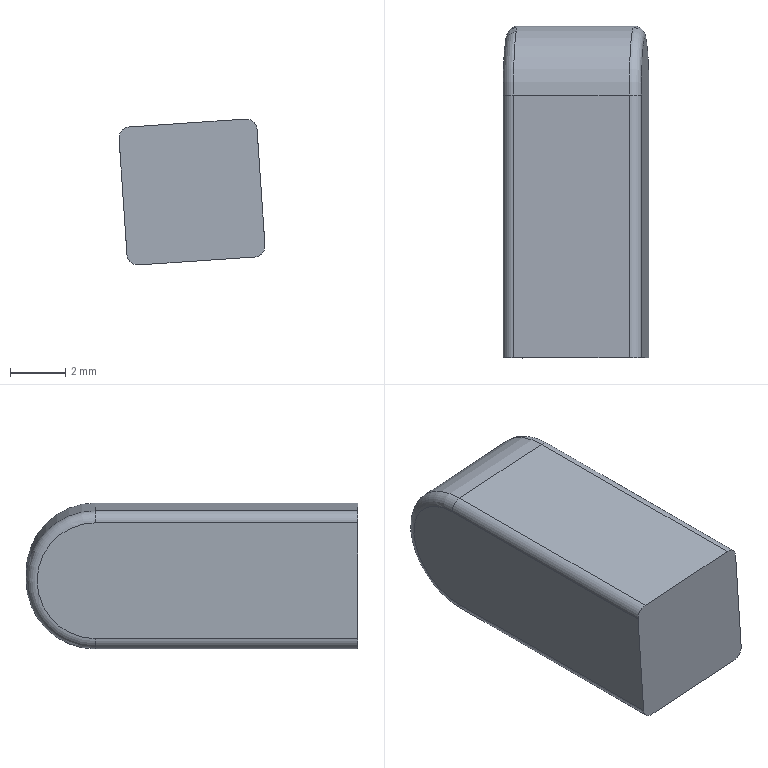Component | SolidWorks | GB_T1096-1979PlainParallelKeyC-type5_12-2 | 1 solid | 13 faces | box 5.28 x 12 x 5.28 mm | volume 285 mm3 | cylinder 6 | plane 5 | torus 2 | commonest cylinder face diameters 0.8 x4 5 x2
build123d program:
from build123d import *

# Parameters (mm, degrees)
BASE_EXTRUDE_DEPTH = 5
FILLET1_R          = 0.4


with BuildPart() as part:
    # Sketch1 → Base-Extrude (new body)
    with BuildSketch(Plane.XY):
        with BuildLine():
            Line((-9, 2.5), (0.5, 2.5))
            Line((0.5, 2.5), (0.5, -2.5))
            Line((0.5, -2.5), (-9, -2.5))
            ThreePointArc((-9, -2.5), (-11.5, 0), (-9, 2.5))
        make_face()
    extrude(amount=BASE_EXTRUDE_DEPTH)

    # Fillet1
    fillet1_edges = [part.edges().sort_by_distance(p)[0] for p in [
        (-11.5, 0, 5),
        (-4.25, -2.5, 5),
        (-4.25, -2.5, 0),
        (-11.5, 0, 0),
        (-4.25, 2.5, 0),
        (-4.25, 2.5, 5),
    ]]
    fillet(fillet1_edges, radius=FILLET1_R)


solid = part.part

# Placed as in the assembly
solid = solid.moved(Location((-17.866, 61.766, -165.86), (180, -86.093, 90)))
STEP:
#1=COLOUR_RGB('',0.7922,0.8196,0.9333);
#2=FILL_AREA_STYLE_COLOUR('',#1);
#3=FILL_AREA_STYLE('',(#2));
#4=SURFACE_STYLE_FILL_AREA(#3);
#5=SURFACE_SIDE_STYLE('',(#4));
#6=SURFACE_STYLE_USAGE(.BOTH.,#5);
#7=PRESENTATION_STYLE_ASSIGNMENT((#6));
#8=CARTESIAN_POINT('',(-0.8774,2.786,-6.64));
#9=VERTEX_POINT('',#8);
#10=CARTESIAN_POINT('',(-0.8841,2.884,-6.542));
#11=VERTEX_POINT('',#10);
#12=CARTESIAN_POINT('',(-0.8841,2.786,-6.542));
#13=DIRECTION('',(0.9977,0.,0.06814));
#14=DIRECTION('',(0.,-1.,0.));
#15=AXIS2_PLACEMENT_3D('',#12,#13,#14);
#16=CIRCLE('',#15,0.09843);
#17=EDGE_CURVE('',#9,#11,#16,.T.);
#18=ORIENTED_EDGE('',*,*,#17,.T.);
#19=CARTESIAN_POINT('',(-0.7191,2.884,-6.531));
#20=VERTEX_POINT('',#19);
#21=CARTESIAN_POINT('',(-0.8998,2.884,-6.543));
#22=DIRECTION('',(0.9977,0.,0.06814));
#23=VECTOR('',#22,39.37);
#24=LINE('',#21,#23);
#25=EDGE_CURVE('',#11,#20,#24,.T.);
#26=ORIENTED_EDGE('',*,*,#25,.T.);
#27=CARTESIAN_POINT('',(-0.7124,2.786,-6.629));
#28=VERTEX_POINT('',#27);
#29=CARTESIAN_POINT('',(-0.7191,2.786,-6.531));
#30=DIRECTION('',(-0.9977,-0.,-0.06814));
#31=DIRECTION('',(0.,-1.,0.));
#32=AXIS2_PLACEMENT_3D('',#29,#30,#31);
#33=CIRCLE('',#32,0.09843);
#34=EDGE_CURVE('',#20,#28,#33,.T.);
#35=ORIENTED_EDGE('',*,*,#34,.T.);
#36=CARTESIAN_POINT('',(-0.8931,2.786,-6.642));
#37=DIRECTION('',(0.9977,0.,0.06814));
#38=VECTOR('',#37,39.37);
#39=LINE('',#36,#38);
#40=EDGE_CURVE('',#9,#28,#39,.T.);
#41=ORIENTED_EDGE('',*,*,#40,.F.);
#42=EDGE_LOOP('',(#18,#26,#35,#41));
#43=FACE_OUTER_BOUND('',#42,.T.);
#44=CARTESIAN_POINT('',(-0.8998,2.786,-6.543));
#45=DIRECTION('',(0.9977,0.,0.06814));
#46=DIRECTION('',(0.,1.,0.));
#47=AXIS2_PLACEMENT_3D('',#44,#45,#46);
#48=CYLINDRICAL_SURFACE('',#47,0.09843);
#49=ADVANCED_FACE('',(#43),#48,.T.);
#50=CARTESIAN_POINT('',(-0.8942,2.412,-6.626));
#51=VERTEX_POINT('',#50);
#52=CARTESIAN_POINT('',(-0.9054,2.412,-6.461));
#53=VERTEX_POINT('',#52);
#54=CARTESIAN_POINT('',(-0.9065,2.412,-6.445));
#55=DIRECTION('',(-0.06814,0.,0.9977));
#56=VECTOR('',#55,39.37);
#57=LINE('',#54,#56);
#58=EDGE_CURVE('',#51,#53,#57,.T.);
#59=ORIENTED_EDGE('',*,*,#58,.F.);
#60=CARTESIAN_POINT('',(-0.8774,2.412,-6.64));
#61=VERTEX_POINT('',#60);
#62=CARTESIAN_POINT('',(-0.8785,2.412,-6.625));
#63=DIRECTION('',(0.,-1.,0.));
#64=DIRECTION('',(-0.9977,0.,-0.06814));
#65=AXIS2_PLACEMENT_3D('',#62,#63,#64);
#66=CIRCLE('',#65,0.01575);
#67=EDGE_CURVE('',#51,#61,#66,.T.);
#68=ORIENTED_EDGE('',*,*,#67,.T.);
#69=CARTESIAN_POINT('',(-0.7124,2.412,-6.629));
#70=VERTEX_POINT('',#69);
#71=CARTESIAN_POINT('',(-0.8931,2.412,-6.642));
#72=DIRECTION('',(0.9977,0.,0.06814));
#73=VECTOR('',#72,39.37);
#74=LINE('',#71,#73);
#75=EDGE_CURVE('',#61,#70,#74,.T.);
#76=ORIENTED_EDGE('',*,*,#75,.T.);
#77=CARTESIAN_POINT('',(-0.6978,2.412,-6.612));
#78=VERTEX_POINT('',#77);
#79=CARTESIAN_POINT('',(-0.7135,2.412,-6.613));
#80=DIRECTION('',(0.,-1.,0.));
#81=DIRECTION('',(-0.9977,0.,-0.06814));
#82=AXIS2_PLACEMENT_3D('',#79,#80,#81);
#83=CIRCLE('',#82,0.01575);
#84=EDGE_CURVE('',#70,#78,#83,.T.);
#85=ORIENTED_EDGE('',*,*,#84,.T.);
#86=CARTESIAN_POINT('',(-0.709,2.412,-6.447));
#87=VERTEX_POINT('',#86);
#88=CARTESIAN_POINT('',(-0.7101,2.412,-6.432));
#89=DIRECTION('',(-0.06814,0.,0.9977));
#90=VECTOR('',#89,39.37);
#91=LINE('',#88,#90);
#92=EDGE_CURVE('',#78,#87,#91,.T.);
#93=ORIENTED_EDGE('',*,*,#92,.T.);
#94=CARTESIAN_POINT('',(-0.7258,2.412,-6.433));
#95=VERTEX_POINT('',#94);
#96=CARTESIAN_POINT('',(-0.7247,2.412,-6.449));
#97=DIRECTION('',(0.,-1.,0.));
#98=DIRECTION('',(-0.9977,0.,-0.06814));
#99=AXIS2_PLACEMENT_3D('',#96,#97,#98);
#100=CIRCLE('',#99,0.01575);
#101=EDGE_CURVE('',#87,#95,#100,.T.);
#102=ORIENTED_EDGE('',*,*,#101,.T.);
#103=CARTESIAN_POINT('',(-0.8908,2.412,-6.444));
#104=VERTEX_POINT('',#103);
#105=CARTESIAN_POINT('',(-0.9065,2.412,-6.445));
#106=DIRECTION('',(0.9977,0.,0.06814));
#107=VECTOR('',#106,39.37);
#108=LINE('',#105,#107);
#109=EDGE_CURVE('',#104,#95,#108,.T.);
#110=ORIENTED_EDGE('',*,*,#109,.F.);
#111=CARTESIAN_POINT('',(-0.8897,2.412,-6.46));
#112=DIRECTION('',(0.,-1.,0.));
#113=DIRECTION('',(-0.9977,0.,-0.06814));
#114=AXIS2_PLACEMENT_3D('',#111,#112,#113);
#115=CIRCLE('',#114,0.01575);
#116=EDGE_CURVE('',#104,#53,#115,.T.);
#117=ORIENTED_EDGE('',*,*,#116,.T.);
#118=EDGE_LOOP('',(#59,#68,#76,#85,#93,#102,#110,#117));
#119=FACE_OUTER_BOUND('',#118,.T.);
#120=CARTESIAN_POINT('',(-0.9065,2.412,-6.445));
#121=DIRECTION('',(-0.,1.,-0.));
#122=DIRECTION('',(-0.9977,-0.,-0.06814));
#123=AXIS2_PLACEMENT_3D('',#120,#121,#122);
#124=PLANE('',#123);
#125=ADVANCED_FACE('',(#119),#124,.F.);
#126=CARTESIAN_POINT('',(-0.8908,2.786,-6.444));
#127=VERTEX_POINT('',#126);
#128=CARTESIAN_POINT('',(-0.7258,2.786,-6.433));
#129=VERTEX_POINT('',#128);
#130=CARTESIAN_POINT('',(-0.9065,2.786,-6.445));
#131=DIRECTION('',(0.9977,0.,0.06814));
#132=VECTOR('',#131,39.37);
#133=LINE('',#130,#132);
#134=EDGE_CURVE('',#127,#129,#133,.T.);
#135=ORIENTED_EDGE('',*,*,#134,.F.);
#136=CARTESIAN_POINT('',(-0.8908,2.412,-6.444));
#137=DIRECTION('',(0.,-1.,0.));
#138=VECTOR('',#137,39.37);
#139=LINE('',#136,#138);
#140=EDGE_CURVE('',#127,#104,#139,.T.);
#141=ORIENTED_EDGE('',*,*,#140,.T.);
#142=ORIENTED_EDGE('',*,*,#109,.T.);
#143=CARTESIAN_POINT('',(-0.7258,2.786,-6.433));
#144=DIRECTION('',(-0.,1.,-0.));
#145=VECTOR('',#144,39.37);
#146=LINE('',#143,#145);
#147=EDGE_CURVE('',#95,#129,#146,.T.);
#148=ORIENTED_EDGE('',*,*,#147,.T.);
#149=EDGE_LOOP('',(#135,#141,#142,#148));
#150=FACE_OUTER_BOUND('',#149,.T.);
#151=CARTESIAN_POINT('',(-0.9065,2.786,-6.445));
#152=DIRECTION('',(0.06814,-0.,-0.9977));
#153=DIRECTION('',(0.9977,0.,0.06814));
#154=AXIS2_PLACEMENT_3D('',#151,#152,#153);
#155=PLANE('',#154);
#156=ADVANCED_FACE('',(#150),#155,.F.);
#157=ORIENTED_EDGE('',*,*,#25,.F.);
#158=CARTESIAN_POINT('',(-0.8841,2.786,-6.542));
#159=DIRECTION('',(0.9977,0.,0.06814));
#160=DIRECTION('',(0.,-1.,0.));
#161=AXIS2_PLACEMENT_3D('',#158,#159,#160);
#162=CIRCLE('',#161,0.09843);
#163=EDGE_CURVE('',#11,#127,#162,.T.);
#164=ORIENTED_EDGE('',*,*,#163,.T.);
#165=ORIENTED_EDGE('',*,*,#134,.T.);
#166=CARTESIAN_POINT('',(-0.7191,2.786,-6.531));
#167=DIRECTION('',(-0.9977,-0.,-0.06814));
#168=DIRECTION('',(0.,-1.,0.));
#169=AXIS2_PLACEMENT_3D('',#166,#167,#168);
#170=CIRCLE('',#169,0.09843);
#171=EDGE_CURVE('',#129,#20,#170,.T.);
#172=ORIENTED_EDGE('',*,*,#171,.T.);
#173=EDGE_LOOP('',(#157,#164,#165,#172));
#174=FACE_OUTER_BOUND('',#173,.T.);
#175=CARTESIAN_POINT('',(-0.8998,2.786,-6.543));
#176=DIRECTION('',(0.9977,0.,0.06814));
#177=DIRECTION('',(0.,1.,0.));
#178=AXIS2_PLACEMENT_3D('',#175,#176,#177);
#179=CYLINDRICAL_SURFACE('',#178,0.09843);
#180=ADVANCED_FACE('',(#174),#179,.T.);
#181=ORIENTED_EDGE('',*,*,#75,.F.);
#182=CARTESIAN_POINT('',(-0.8774,2.786,-6.64));
#183=DIRECTION('',(-0.,1.,-0.));
#184=VECTOR('',#183,39.37);
#185=LINE('',#182,#184);
#186=EDGE_CURVE('',#61,#9,#185,.T.);
#187=ORIENTED_EDGE('',*,*,#186,.T.);
#188=ORIENTED_EDGE('',*,*,#40,.T.);
#189=CARTESIAN_POINT('',(-0.7124,2.786,-6.629));
#190=DIRECTION('',(0.,-1.,0.));
#191=VECTOR('',#190,39.37);
#192=LINE('',#189,#191);
#193=EDGE_CURVE('',#28,#70,#192,.T.);
#194=ORIENTED_EDGE('',*,*,#193,.T.);
#195=EDGE_LOOP('',(#181,#187,#188,#194));
#196=FACE_OUTER_BOUND('',#195,.T.);
#197=CARTESIAN_POINT('',(-0.8931,2.786,-6.642));
#198=DIRECTION('',(-0.06814,0.,0.9977));
#199=DIRECTION('',(-0.9977,-0.,-0.06814));
#200=AXIS2_PLACEMENT_3D('',#197,#198,#199);
#201=PLANE('',#200);
#202=ADVANCED_FACE('',(#196),#201,.F.);
#203=CARTESIAN_POINT('',(-0.9054,2.786,-6.461));
#204=VERTEX_POINT('',#203);
#205=CARTESIAN_POINT('',(-0.8942,2.786,-6.626));
#206=VERTEX_POINT('',#205);
#207=CARTESIAN_POINT('',(-0.8998,2.786,-6.543));
#208=DIRECTION('',(-0.9977,-0.,-0.06814));
#209=DIRECTION('',(0.,-1.,0.));
#210=AXIS2_PLACEMENT_3D('',#207,#208,#209);
#211=CIRCLE('',#210,0.08268);
#212=EDGE_CURVE('',#204,#206,#211,.T.);
#213=ORIENTED_EDGE('',*,*,#212,.T.);
#214=CARTESIAN_POINT('',(-0.8942,2.412,-6.626));
#215=DIRECTION('',(0.,-1.,0.));
#216=VECTOR('',#215,39.37);
#217=LINE('',#214,#216);
#218=EDGE_CURVE('',#206,#51,#217,.T.);
#219=ORIENTED_EDGE('',*,*,#218,.T.);
#220=ORIENTED_EDGE('',*,*,#58,.T.);
#221=CARTESIAN_POINT('',(-0.9054,2.786,-6.461));
#222=DIRECTION('',(-0.,1.,-0.));
#223=VECTOR('',#222,39.37);
#224=LINE('',#221,#223);
#225=EDGE_CURVE('',#53,#204,#224,.T.);
#226=ORIENTED_EDGE('',*,*,#225,.T.);
#227=EDGE_LOOP('',(#213,#219,#220,#226));
#228=FACE_OUTER_BOUND('',#227,.T.);
#229=CARTESIAN_POINT('',(-0.8998,2.786,-6.543));
#230=DIRECTION('',(-0.9977,-0.,-0.06814));
#231=DIRECTION('',(0.,-1.,0.));
#232=AXIS2_PLACEMENT_3D('',#229,#230,#231);
#233=PLANE('',#232);
#234=ADVANCED_FACE('',(#228),#233,.T.);
#235=CARTESIAN_POINT('',(-0.6978,2.786,-6.612));
#236=VERTEX_POINT('',#235);
#237=CARTESIAN_POINT('',(-0.709,2.786,-6.447));
#238=VERTEX_POINT('',#237);
#239=CARTESIAN_POINT('',(-0.7034,2.786,-6.53));
#240=DIRECTION('',(0.9977,0.,0.06814));
#241=DIRECTION('',(0.,-1.,0.));
#242=AXIS2_PLACEMENT_3D('',#239,#240,#241);
#243=CIRCLE('',#242,0.08268);
#244=EDGE_CURVE('',#236,#238,#243,.T.);
#245=ORIENTED_EDGE('',*,*,#244,.T.);
#246=CARTESIAN_POINT('',(-0.709,2.786,-6.447));
#247=DIRECTION('',(0.,-1.,0.));
#248=VECTOR('',#247,39.37);
#249=LINE('',#246,#248);
#250=EDGE_CURVE('',#238,#87,#249,.T.);
#251=ORIENTED_EDGE('',*,*,#250,.T.);
#252=ORIENTED_EDGE('',*,*,#92,.F.);
#253=CARTESIAN_POINT('',(-0.6978,2.786,-6.612));
#254=DIRECTION('',(-0.,1.,-0.));
#255=VECTOR('',#254,39.37);
#256=LINE('',#253,#255);
#257=EDGE_CURVE('',#78,#236,#256,.T.);
#258=ORIENTED_EDGE('',*,*,#257,.T.);
#259=EDGE_LOOP('',(#245,#251,#252,#258));
#260=FACE_OUTER_BOUND('',#259,.T.);
#261=CARTESIAN_POINT('',(-0.7034,2.786,-6.53));
#262=DIRECTION('',(-0.9977,-0.,-0.06814));
#263=DIRECTION('',(0.,-1.,0.));
#264=AXIS2_PLACEMENT_3D('',#261,#262,#263);
#265=PLANE('',#264);
#266=ADVANCED_FACE('',(#260),#265,.F.);
#267=ORIENTED_EDGE('',*,*,#116,.F.);
#268=ORIENTED_EDGE('',*,*,#140,.F.);
#269=CARTESIAN_POINT('',(-0.8897,2.786,-6.46));
#270=DIRECTION('',(-0.,1.,-0.));
#271=DIRECTION('',(-0.9977,0.,-0.06814));
#272=AXIS2_PLACEMENT_3D('',#269,#270,#271);
#273=CIRCLE('',#272,0.01575);
#274=EDGE_CURVE('',#204,#127,#273,.T.);
#275=ORIENTED_EDGE('',*,*,#274,.F.);
#276=ORIENTED_EDGE('',*,*,#225,.F.);
#277=EDGE_LOOP('',(#267,#268,#275,#276));
#278=FACE_OUTER_BOUND('',#277,.T.);
#279=CARTESIAN_POINT('',(-0.8897,2.786,-6.46));
#280=DIRECTION('',(0.,-1.,0.));
#281=DIRECTION('',(0.9977,0.,0.06814));
#282=AXIS2_PLACEMENT_3D('',#279,#280,#281);
#283=CYLINDRICAL_SURFACE('',#282,0.01575);
#284=ADVANCED_FACE('',(#278),#283,.T.);
#285=ORIENTED_EDGE('',*,*,#274,.T.);
#286=ORIENTED_EDGE('',*,*,#163,.F.);
#287=ORIENTED_EDGE('',*,*,#17,.F.);
#288=CARTESIAN_POINT('',(-0.8785,2.786,-6.625));
#289=DIRECTION('',(0.,-1.,0.));
#290=DIRECTION('',(0.9977,0.,0.06814));
#291=AXIS2_PLACEMENT_3D('',#288,#289,#290);
#292=CIRCLE('',#291,0.01575);
#293=EDGE_CURVE('',#206,#9,#292,.T.);
#294=ORIENTED_EDGE('',*,*,#293,.F.);
#295=ORIENTED_EDGE('',*,*,#212,.F.);
#296=EDGE_LOOP('',(#285,#286,#287,#294,#295));
#297=FACE_OUTER_BOUND('',#296,.T.);
#298=CARTESIAN_POINT('',(-0.8841,2.786,-6.542));
#299=DIRECTION('',(-0.9977,-0.,-0.06814));
#300=DIRECTION('',(0.,-1.,0.));
#301=AXIS2_PLACEMENT_3D('',#298,#299,#300);
#302=TOROIDAL_SURFACE('',#301,0.08268,0.01575);
#303=ADVANCED_FACE('',(#297),#302,.T.);
#304=ORIENTED_EDGE('',*,*,#293,.T.);
#305=ORIENTED_EDGE('',*,*,#186,.F.);
#306=ORIENTED_EDGE('',*,*,#67,.F.);
#307=ORIENTED_EDGE('',*,*,#218,.F.);
#308=EDGE_LOOP('',(#304,#305,#306,#307));
#309=FACE_OUTER_BOUND('',#308,.T.);
#310=CARTESIAN_POINT('',(-0.8785,2.786,-6.625));
#311=DIRECTION('',(-0.,1.,-0.));
#312=DIRECTION('',(-0.9977,0.,-0.06814));
#313=AXIS2_PLACEMENT_3D('',#310,#311,#312);
#314=CYLINDRICAL_SURFACE('',#313,0.01575);
#315=ADVANCED_FACE('',(#309),#314,.T.);
#316=ORIENTED_EDGE('',*,*,#84,.F.);
#317=ORIENTED_EDGE('',*,*,#193,.F.);
#318=CARTESIAN_POINT('',(-0.7135,2.786,-6.613));
#319=DIRECTION('',(-0.,1.,-0.));
#320=DIRECTION('',(-0.9977,0.,-0.06814));
#321=AXIS2_PLACEMENT_3D('',#318,#319,#320);
#322=CIRCLE('',#321,0.01575);
#323=EDGE_CURVE('',#236,#28,#322,.T.);
#324=ORIENTED_EDGE('',*,*,#323,.F.);
#325=ORIENTED_EDGE('',*,*,#257,.F.);
#326=EDGE_LOOP('',(#316,#317,#324,#325));
#327=FACE_OUTER_BOUND('',#326,.T.);
#328=CARTESIAN_POINT('',(-0.7135,2.786,-6.613));
#329=DIRECTION('',(0.,-1.,0.));
#330=DIRECTION('',(0.9977,0.,0.06814));
#331=AXIS2_PLACEMENT_3D('',#328,#329,#330);
#332=CYLINDRICAL_SURFACE('',#331,0.01575);
#333=ADVANCED_FACE('',(#327),#332,.T.);
#334=ORIENTED_EDGE('',*,*,#323,.T.);
#335=ORIENTED_EDGE('',*,*,#34,.F.);
#336=ORIENTED_EDGE('',*,*,#171,.F.);
#337=CARTESIAN_POINT('',(-0.7247,2.786,-6.449));
#338=DIRECTION('',(0.,-1.,0.));
#339=DIRECTION('',(0.9977,0.,0.06814));
#340=AXIS2_PLACEMENT_3D('',#337,#338,#339);
#341=CIRCLE('',#340,0.01575);
#342=EDGE_CURVE('',#238,#129,#341,.T.);
#343=ORIENTED_EDGE('',*,*,#342,.F.);
#344=ORIENTED_EDGE('',*,*,#244,.F.);
#345=EDGE_LOOP('',(#334,#335,#336,#343,#344));
#346=FACE_OUTER_BOUND('',#345,.T.);
#347=CARTESIAN_POINT('',(-0.7191,2.786,-6.531));
#348=DIRECTION('',(-0.9977,-0.,-0.06814));
#349=DIRECTION('',(0.,-1.,0.));
#350=AXIS2_PLACEMENT_3D('',#347,#348,#349);
#351=TOROIDAL_SURFACE('',#350,0.08268,0.01575);
#352=ADVANCED_FACE('',(#346),#351,.T.);
#353=ORIENTED_EDGE('',*,*,#101,.F.);
#354=ORIENTED_EDGE('',*,*,#250,.F.);
#355=ORIENTED_EDGE('',*,*,#342,.T.);
#356=ORIENTED_EDGE('',*,*,#147,.F.);
#357=EDGE_LOOP('',(#353,#354,#355,#356));
#358=FACE_OUTER_BOUND('',#357,.T.);
#359=CARTESIAN_POINT('',(-0.7247,2.786,-6.449));
#360=DIRECTION('',(-0.,1.,-0.));
#361=DIRECTION('',(-0.9977,0.,-0.06814));
#362=AXIS2_PLACEMENT_3D('',#359,#360,#361);
#363=CYLINDRICAL_SURFACE('',#362,0.01575);
#364=ADVANCED_FACE('',(#358),#363,.T.);
#365=CLOSED_SHELL('',(#49,#125,#156,#180,#202,#234,#266,#284,#303,#315,#333,#352,#364));
#366=MANIFOLD_SOLID_BREP('',#365);
#367=STYLED_ITEM('',(#7),#366);
#368=(LENGTH_UNIT()NAMED_UNIT(*)SI_UNIT($,.METRE.));
#369=LENGTH_MEASURE_WITH_UNIT(LENGTH_MEASURE(0.0254),#368);
#370=DIMENSIONAL_EXPONENTS(1.,0.,0.,0.,0.,0.,0.);
#371=(CONVERSION_BASED_UNIT('',#369)LENGTH_UNIT()NAMED_UNIT(#370));
#372=UNCERTAINTY_MEASURE_WITH_UNIT(LENGTH_MEASURE(0.00001),#371,'','');
#373=(NAMED_UNIT(*)PLANE_ANGLE_UNIT()SI_UNIT($,.RADIAN.));
#374=(NAMED_UNIT(*)SI_UNIT($,.STERADIAN.)SOLID_ANGLE_UNIT());
#375=(GEOMETRIC_REPRESENTATION_CONTEXT(3)GLOBAL_UNCERTAINTY_ASSIGNED_CONTEXT((#372))GLOBAL_UNIT_ASSIGNED_CONTEXT((#371,#373,#374))REPRESENTATION_CONTEXT('',''));
#376=MECHANICAL_DESIGN_GEOMETRIC_PRESENTATION_REPRESENTATION('',(#367),#375);
#377=CARTESIAN_POINT('',(0.,0.,0.));
#378=DIRECTION('',(0.,0.,1.));
#379=DIRECTION('',(1.,0.,0.));
#380=AXIS2_PLACEMENT_3D('',#377,#378,#379);
#381=(LENGTH_UNIT()NAMED_UNIT(*)SI_UNIT($,.METRE.));
#382=LENGTH_MEASURE_WITH_UNIT(LENGTH_MEASURE(0.0254),#381);
#383=DIMENSIONAL_EXPONENTS(1.,0.,0.,0.,0.,0.,0.);
#384=(CONVERSION_BASED_UNIT('',#382)LENGTH_UNIT()NAMED_UNIT(#383));
#385=UNCERTAINTY_MEASURE_WITH_UNIT(LENGTH_MEASURE(0.00001),#384,'','');
#386=(NAMED_UNIT(*)PLANE_ANGLE_UNIT()SI_UNIT($,.RADIAN.));
#387=(NAMED_UNIT(*)SI_UNIT($,.STERADIAN.)SOLID_ANGLE_UNIT());
#388=(GEOMETRIC_REPRESENTATION_CONTEXT(3)GLOBAL_UNCERTAINTY_ASSIGNED_CONTEXT((#385))GLOBAL_UNIT_ASSIGNED_CONTEXT((#384,#386,#387))REPRESENTATION_CONTEXT('',''));
#389=ADVANCED_BREP_SHAPE_REPRESENTATION('',(#366,#380),#388);
#390=PRESENTATION_LAYER_ASSIGNMENT('','',(#367));